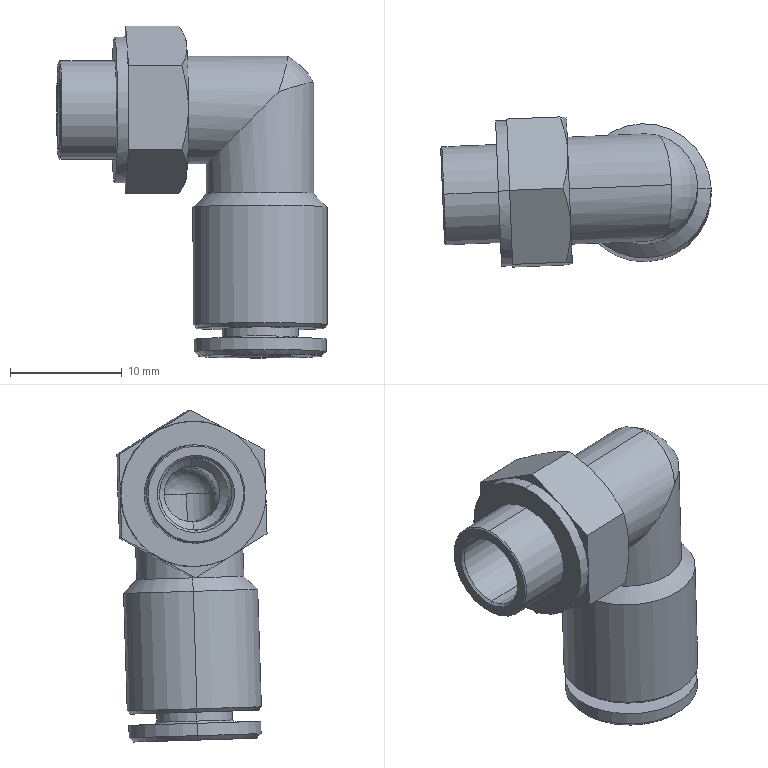Component | SolidWorks | NPQH-L-G18-Q6-P10-1 | 1 solid | 66 faces | volume 2732 mm3 | cone 23 | cylinder 22 | plane 19 | torus 1 | spline 1 | commonest cylinder face diameters 9.6 x4 5 x4 8.8 x2 12 x2 6.8 x2 11.8 x2 13 x2 6 x2